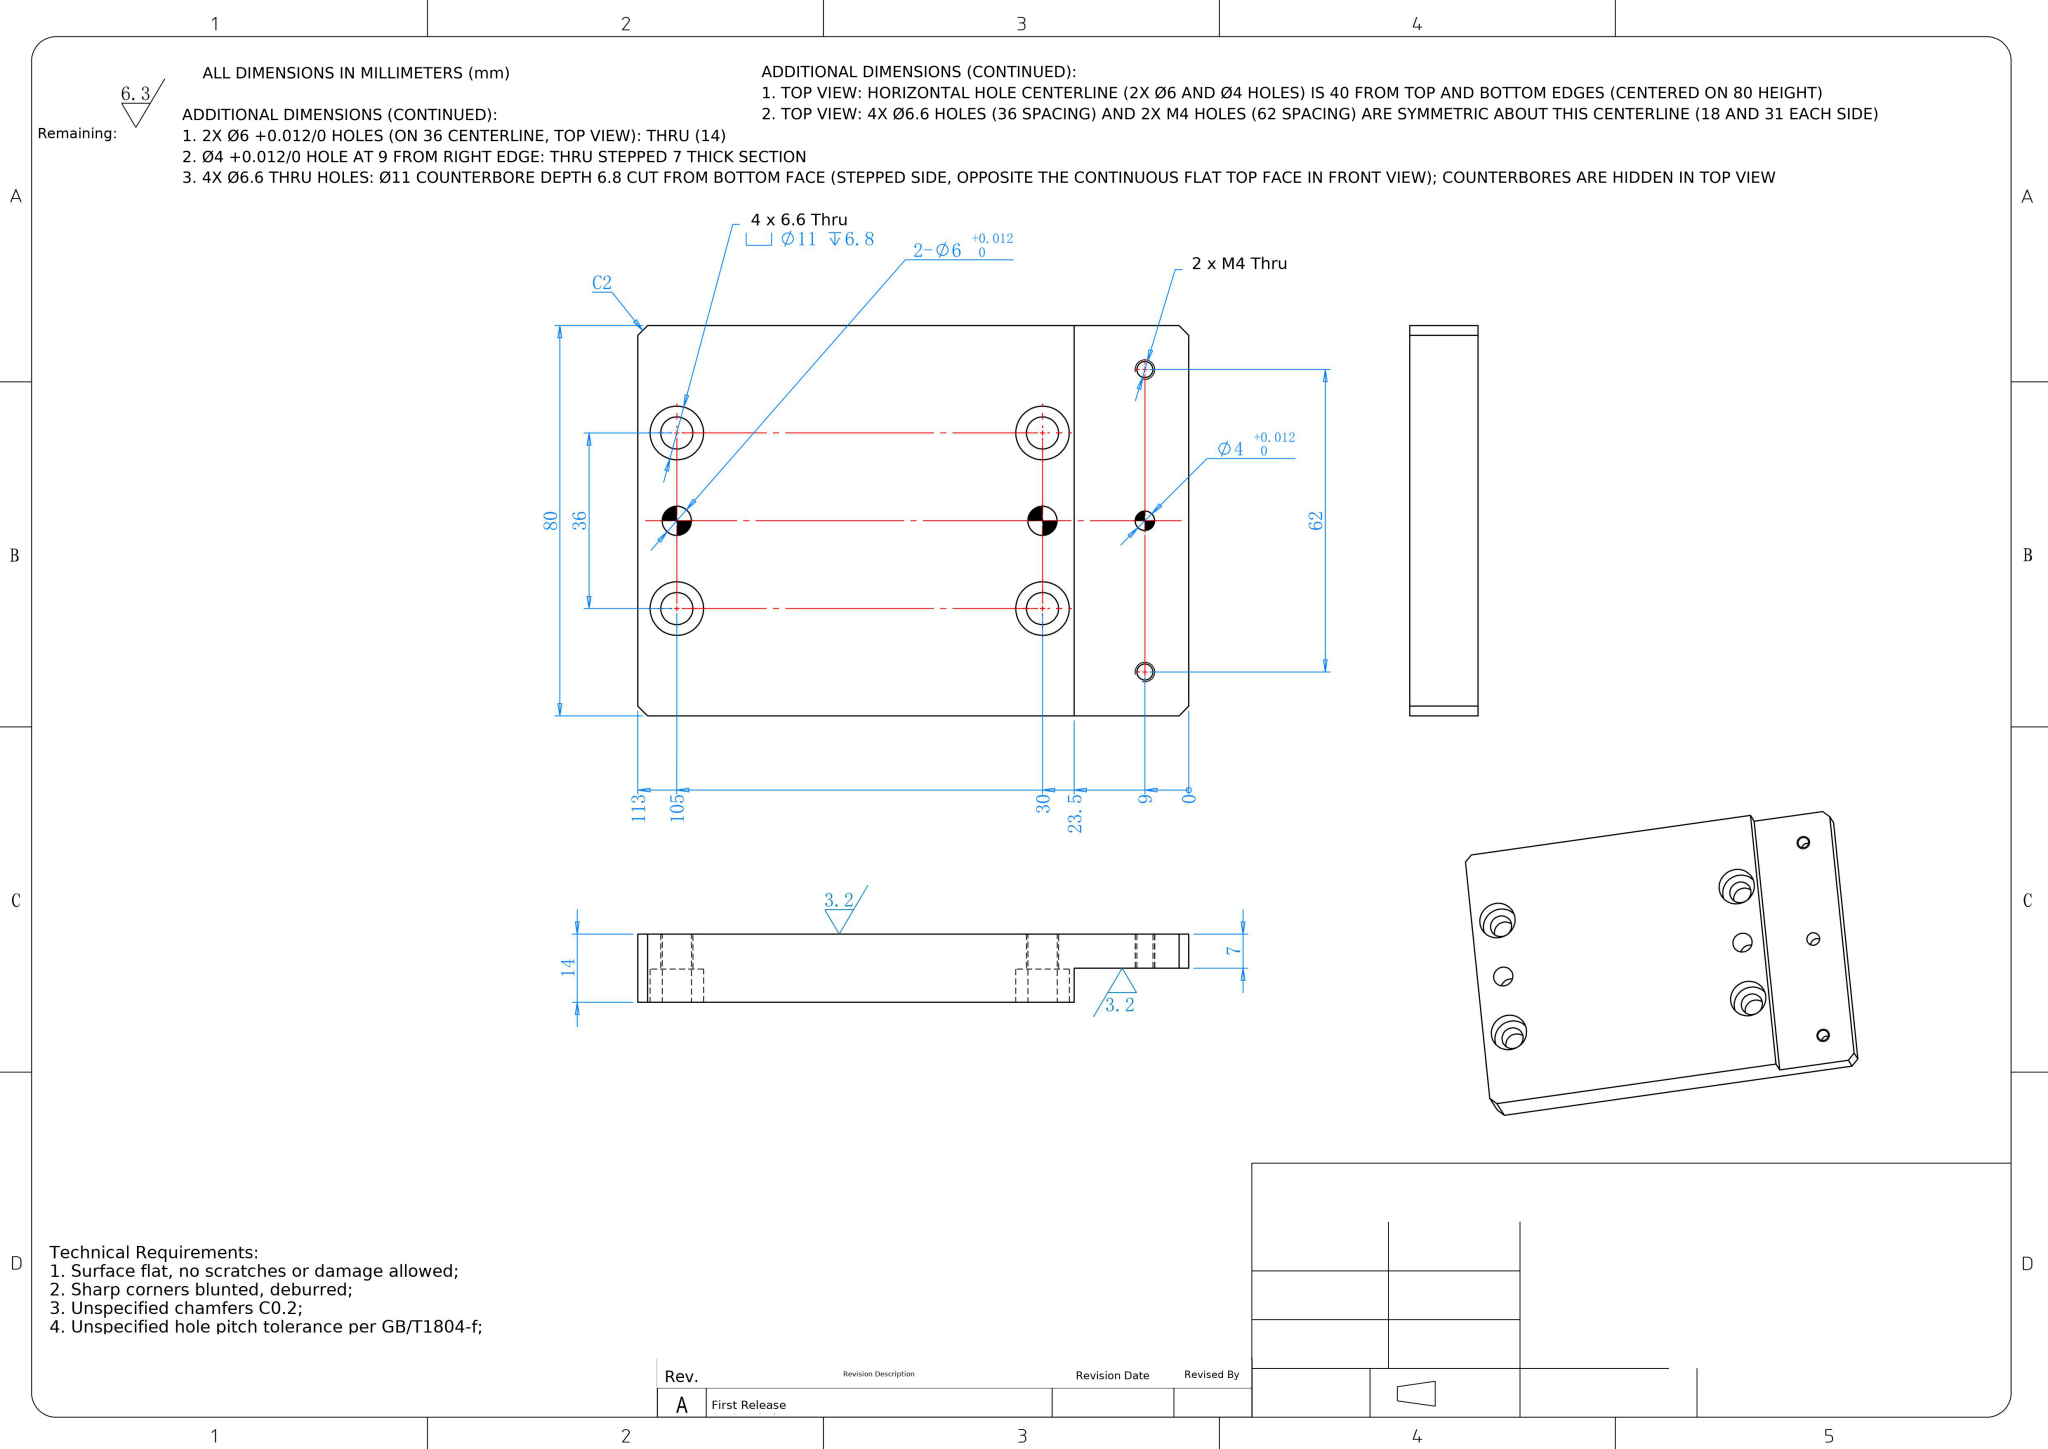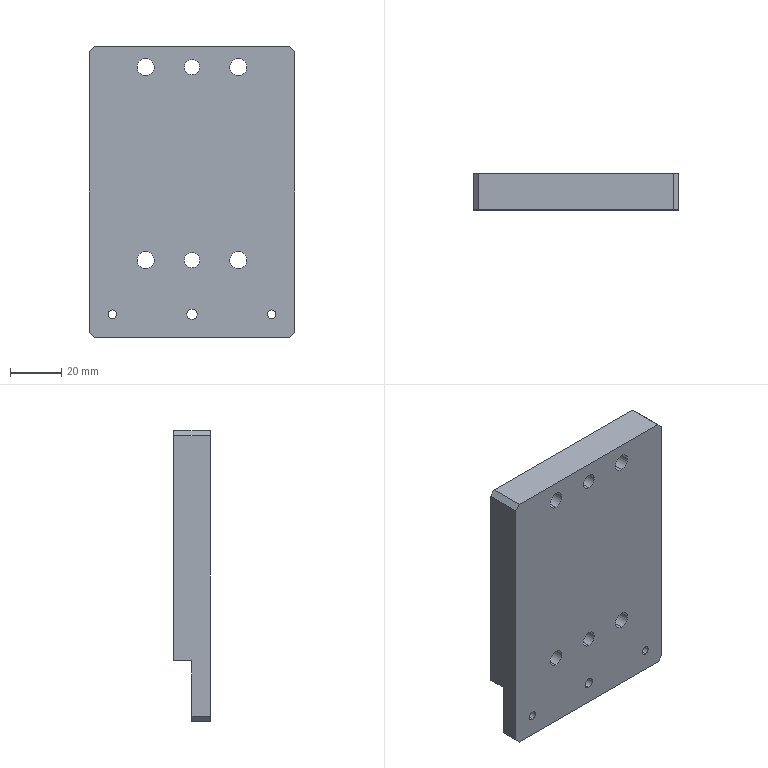Part | NX | mm | 1 solid | 42 faces | box 80 x 14 x 113 mm | volume 108746 mm3 | cylinder 26 | plane 16 | commonest cylinder face diameters 11 x8 6.6 x8 3.3 x4 6 x4 4 x2